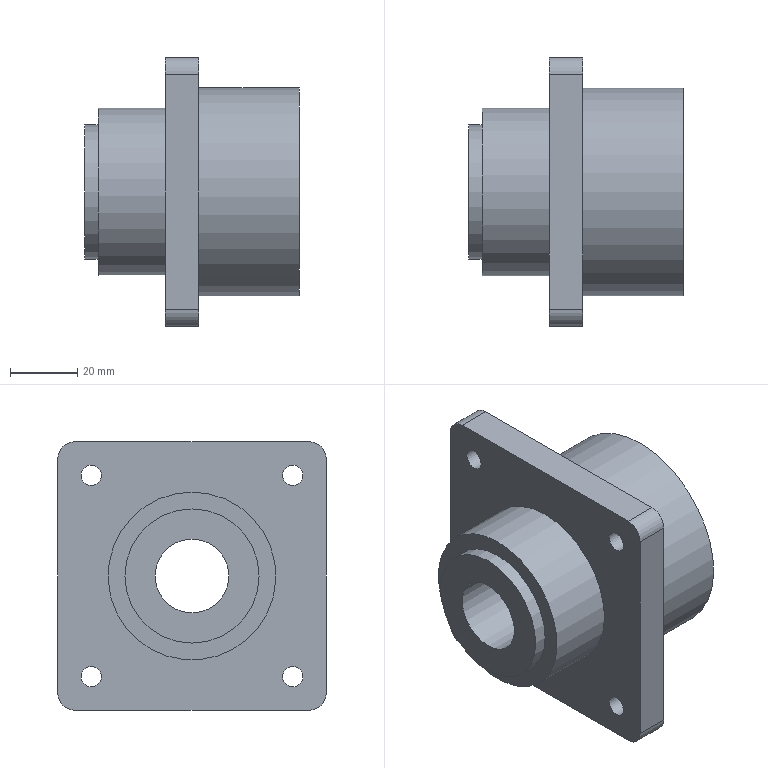Component | NX | VALVE_SEAT | 1 solid | 25 faces | volume 142420 mm3 | cylinder 14 | plane 11 | commonest cylinder face diameters 6 x4 10 x4 22 x1 50 x1 40 x1 42 x1 62 x1 45 x1